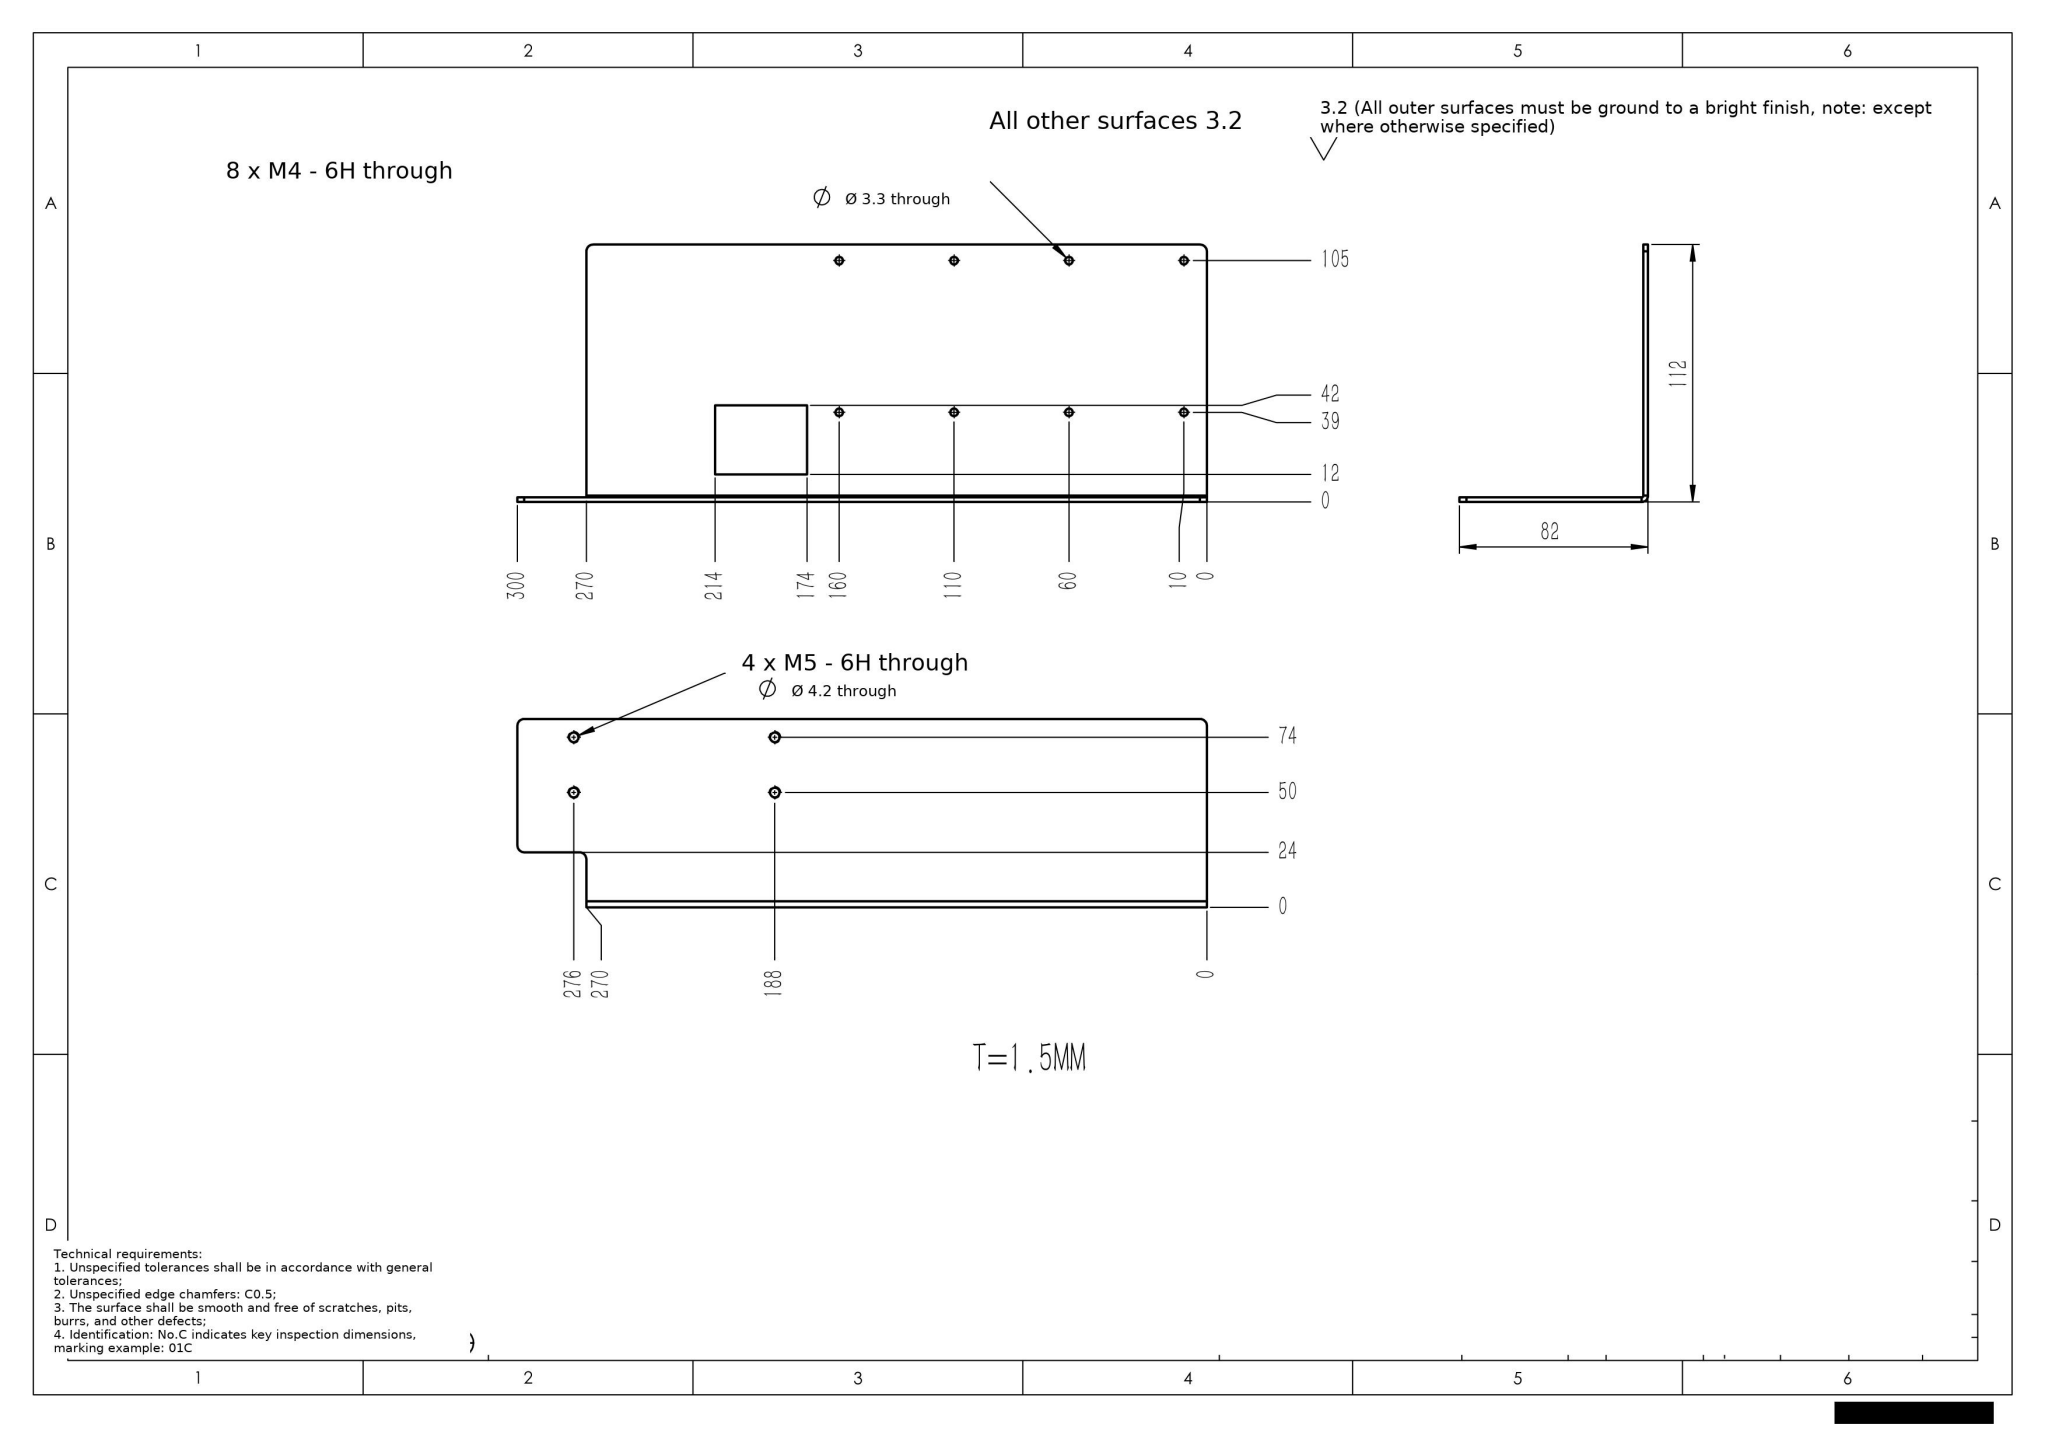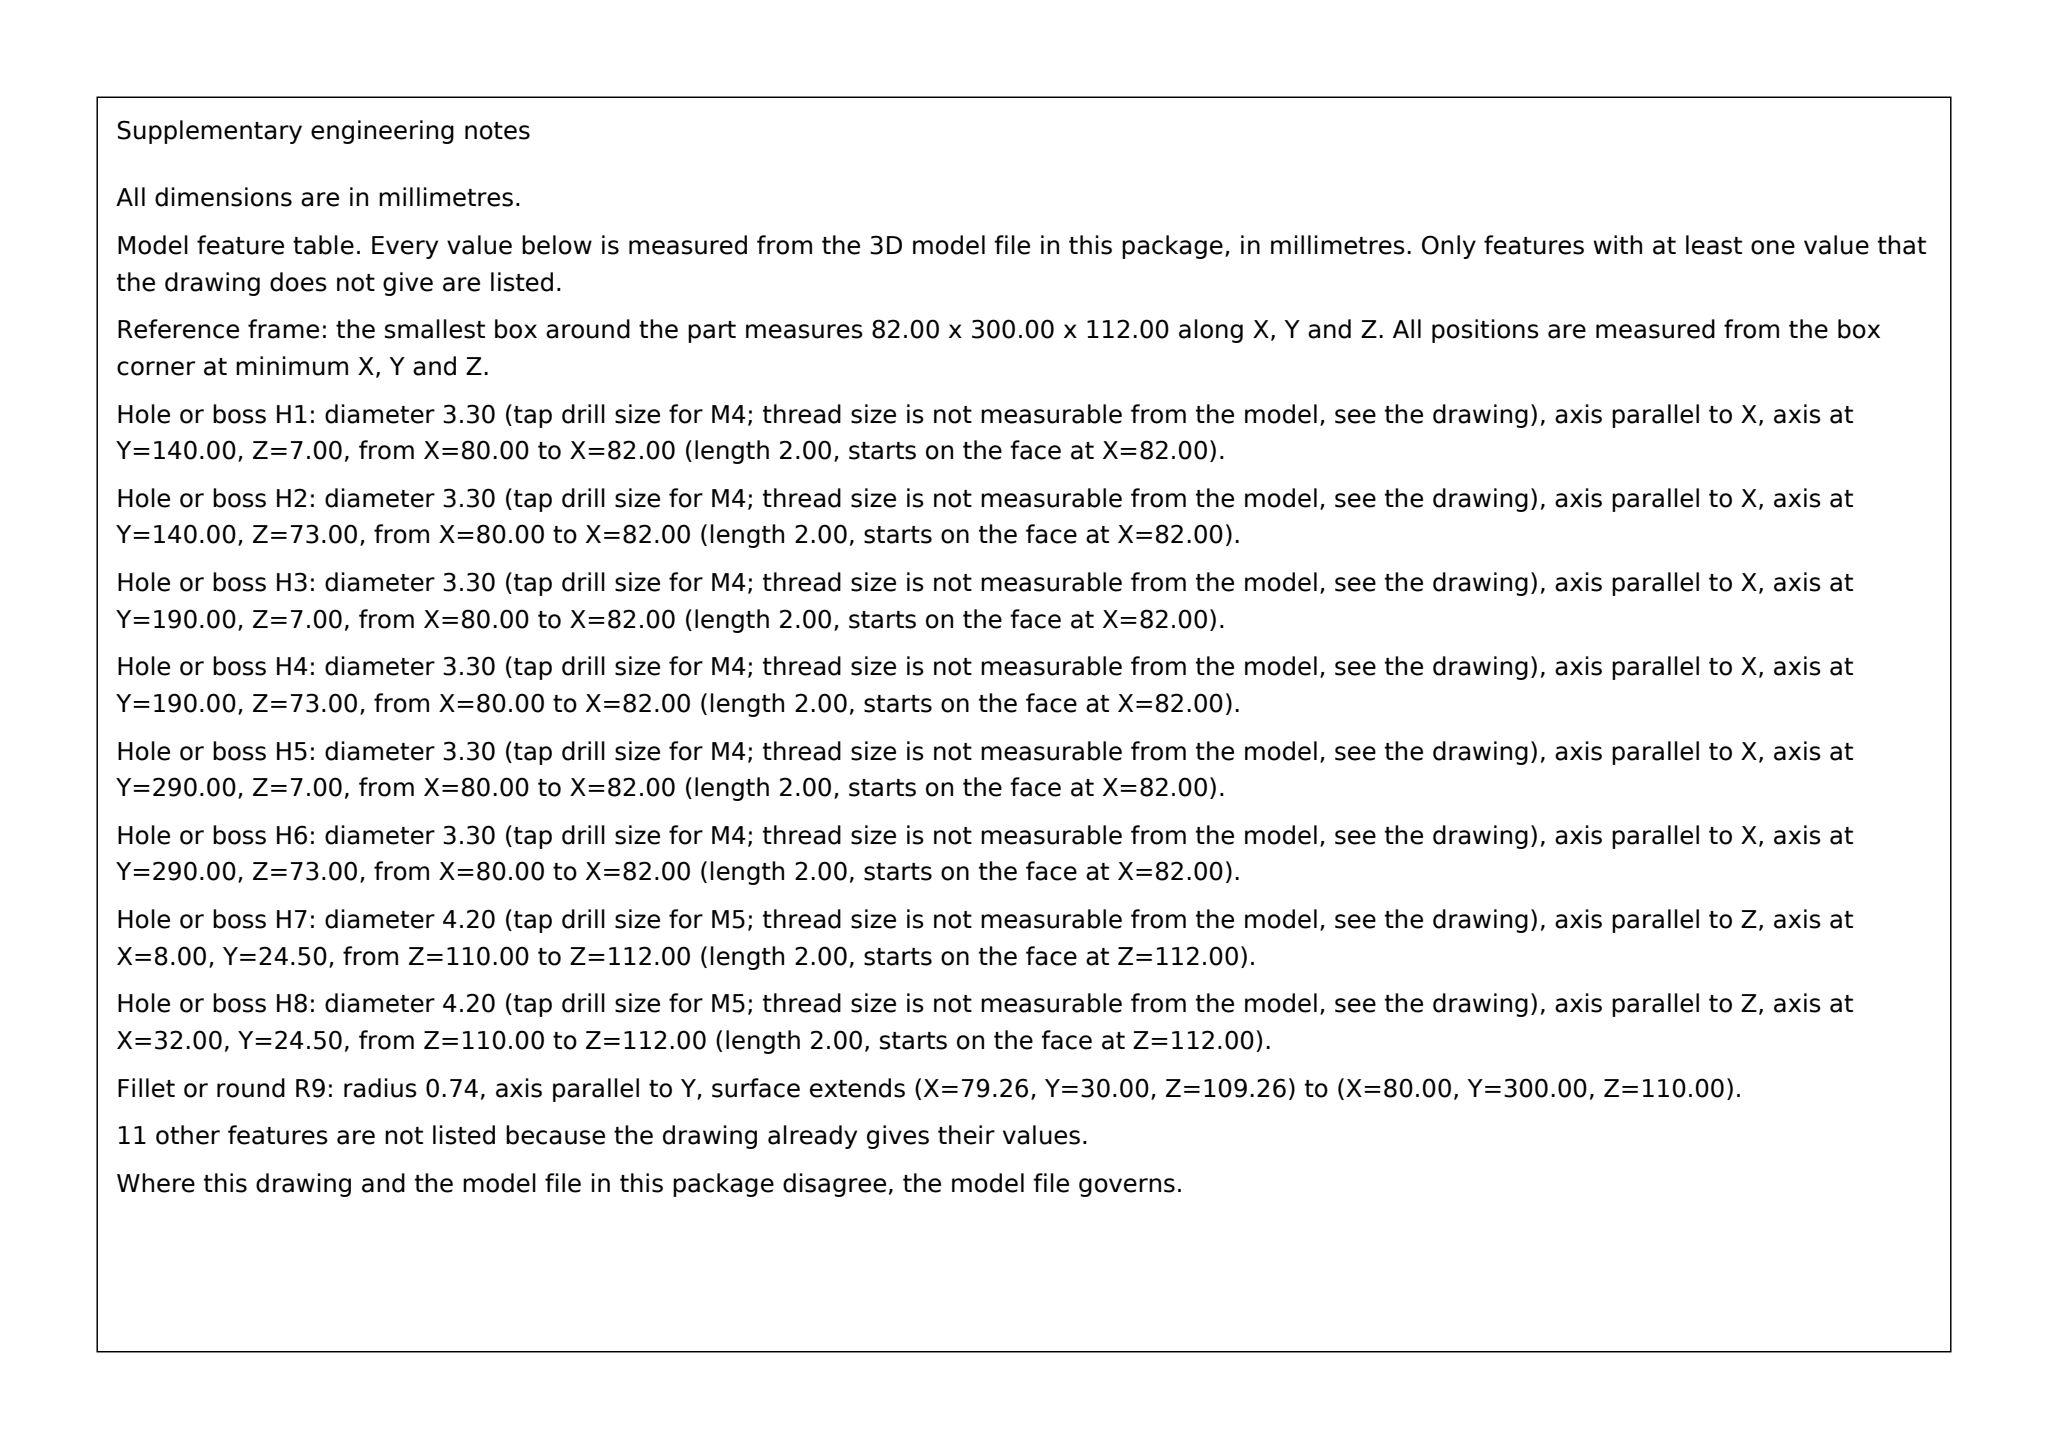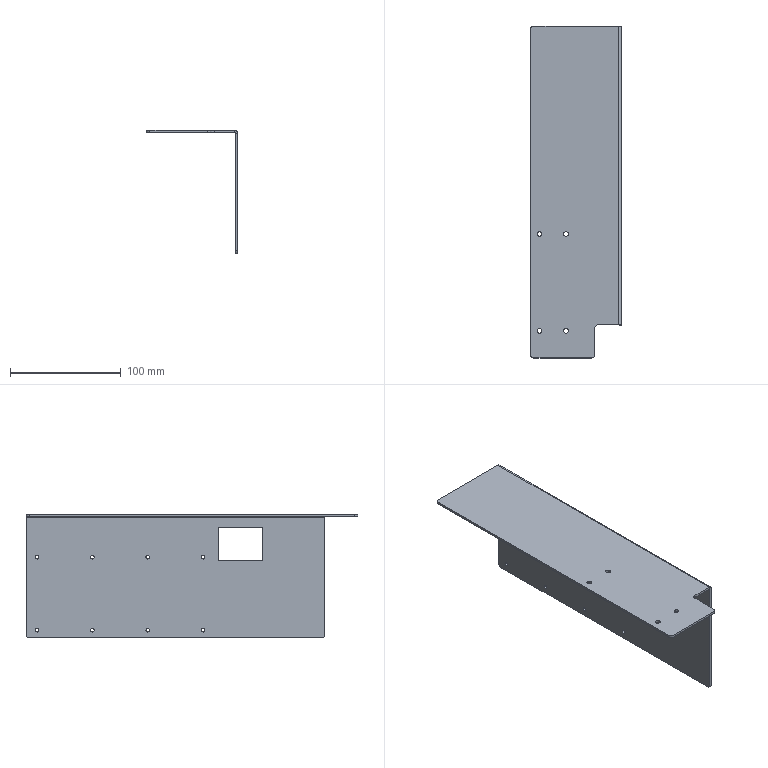Part | SolidWorks | mm | 1 solid | 50 faces | box 82 x 300 x 112 mm | volume 104094 mm3 | cylinder 32 | plane 18 | commonest cylinder face diameters 3.3 x16 4.2 x8 6 x6 1.473 x1 5.473 x1